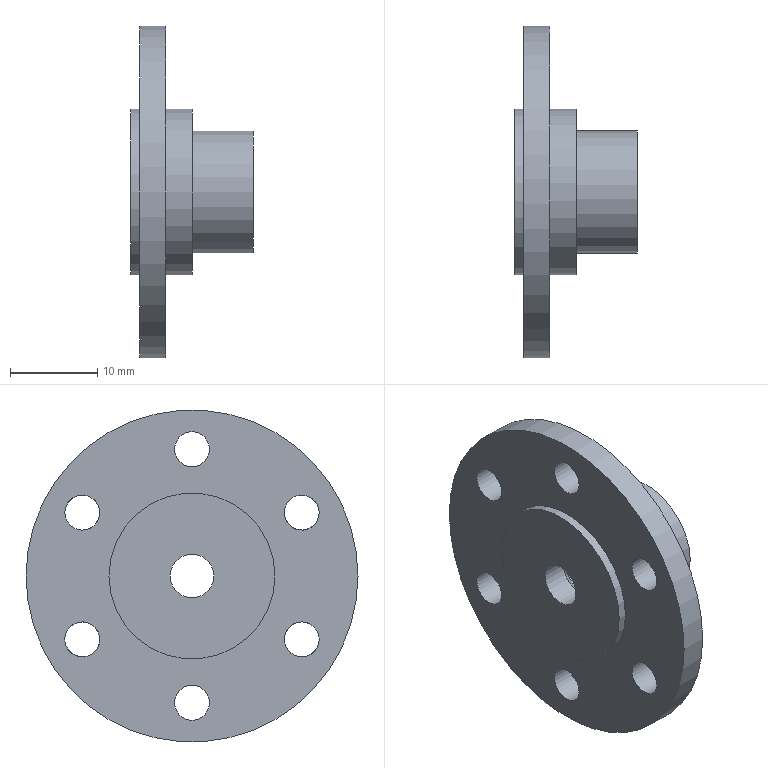Component | NX | FRONT_END_COVER_2 | 1 solid | 19 faces | volume 4515 mm3 | cylinder 12 | plane 6 | cone 1 | commonest cylinder face diameters 4 x6 19 x2 38 x1 14 x1 10 x1 5 x1